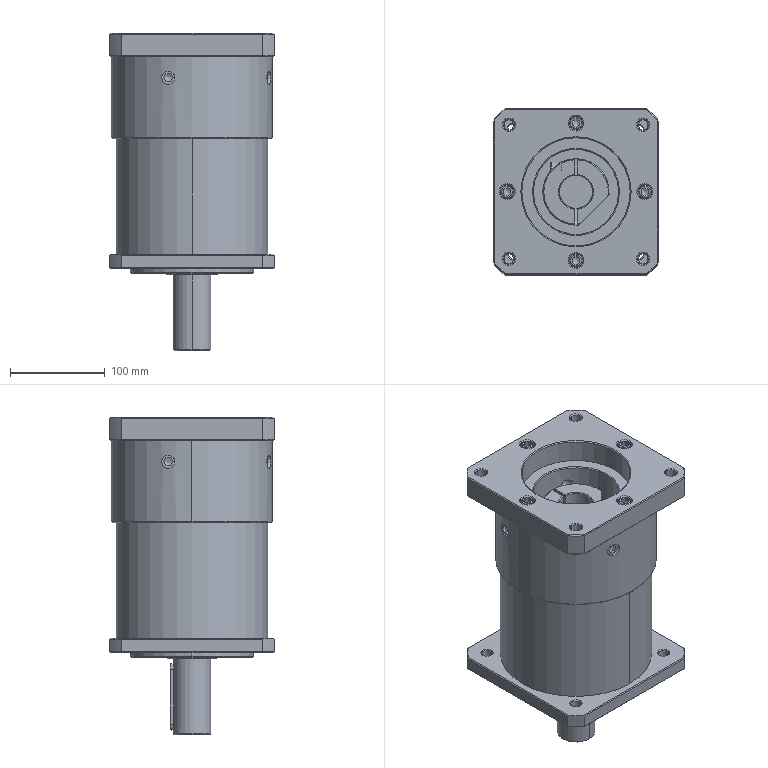Component | SolidWorks | PlanetaryReducer-PLF142-1 | 1 solid | 457 faces | volume 5253611 mm3 | plane 211 | cylinder 133 | cone 94 | spline 19 | commonest cylinder face diameters 13.5 x24 14 x24 12 x21 15 x21 11 x8 230 x8 70 x3 40 x2